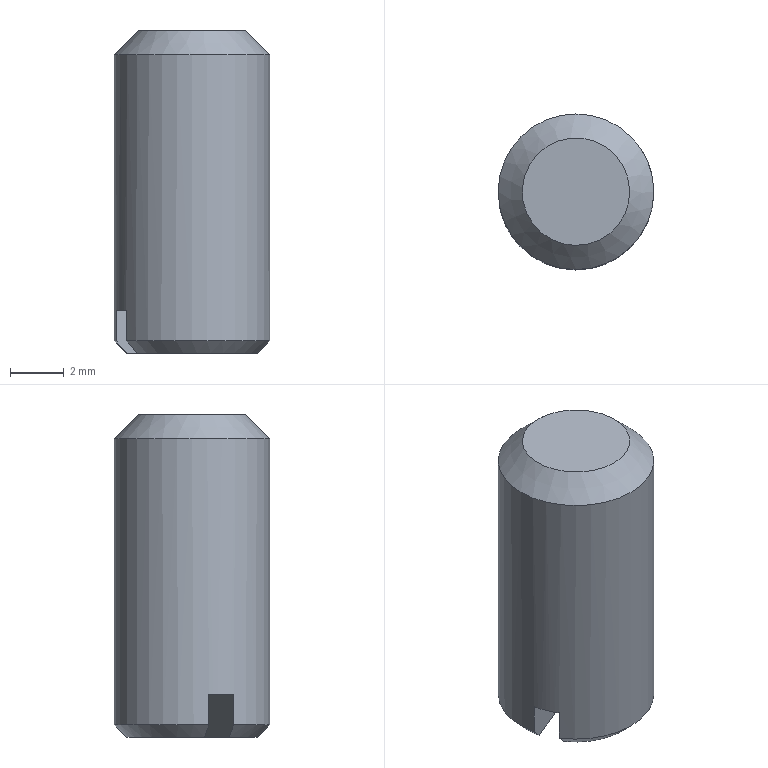Component | NX | GB73-85_M6X12 | 1 solid | 10 faces | box 5.8 x 5.8 x 12 mm | volume 299 mm3 | plane 6 | cone 3 | cylinder 1 | commonest cylinder face diameters 5.795 x1
STEP:
#1=CARTESIAN_POINT('',(0.,0.,0.));
#2=DIRECTION('',(0.,0.,1.));
#3=DIRECTION('',(1.,0.,0.));
#4=AXIS2_PLACEMENT_3D('',#1,#2,#3);
#5=CARTESIAN_POINT('',(-0.3824,57.675,-48.328));
#6=VERTEX_POINT('',#5);
#7=CARTESIAN_POINT('',(4.04,59.509,-48.328));
#8=VERTEX_POINT('',#7);
#9=CARTESIAN_POINT('',(-3.524,56.372,-48.328));
#10=DIRECTION('',(0.9237,0.383,0.));
#11=VECTOR('',#10,1.);
#12=LINE('',#9,#11);
#13=CARTESIAN_POINT('',(1.084,60.389,-48.328));
#14=DIRECTION('',(0.,0.,1.));
#15=DIRECTION('',(0.9237,0.383,0.));
#16=AXIS2_PLACEMENT_3D('',#13,#14,#15);
#17=PLANE('',#16);
#18=CARTESIAN_POINT('',(-5.795,-1.946));
#19=DIRECTION('',(1.,0.));
#20=VECTOR('',#19,1.);
#21=LINE('',#18,#20);
#22=(GEOMETRIC_REPRESENTATION_CONTEXT(2)PARAMETRIC_REPRESENTATION_CONTEXT()REPRESENTATION_CONTEXT('',''));
#23=DEFINITIONAL_REPRESENTATION('',(#21),#22);
#24=PCURVE('',#17,#23);
#25=CARTESIAN_POINT('',(-3.524,56.372,-48.328));
#26=DIRECTION('',(-0.383,0.9237,-0.));
#27=DIRECTION('',(0.,-0.,-1.));
#28=AXIS2_PLACEMENT_3D('',#25,#26,#27);
#29=PLANE('',#28);
#30=CARTESIAN_POINT('',(0.,0.));
#31=DIRECTION('',(0.,-1.));
#32=VECTOR('',#31,1.);
#33=LINE('',#30,#32);
#34=(GEOMETRIC_REPRESENTATION_CONTEXT(2)PARAMETRIC_REPRESENTATION_CONTEXT()REPRESENTATION_CONTEXT('',''));
#35=DEFINITIONAL_REPRESENTATION('',(#33),#34);
#36=PCURVE('',#29,#35);
#37=SURFACE_CURVE('',#12,(#24,#36),.PCURVE_S1.);
#38=EDGE_CURVE('',#6,#8,#37,.T.);
#39=ORIENTED_EDGE('',*,*,#38,.F.);
#40=CARTESIAN_POINT('',(2.02,58.13,-48.328));
#41=DIRECTION('',(0.,0.,-1.));
#42=DIRECTION('',(-0.9237,-0.383,0.));
#43=AXIS2_PLACEMENT_3D('',#40,#41,#42);
#44=CIRCLE('',#43,2.446);
#45=CARTESIAN_POINT('',(-2.446,-2.446));
#46=CARTESIAN_POINT('',(-2.446,1.79));
#47=CARTESIAN_POINT('',(1.223,-0.3276));
#48=CARTESIAN_POINT('',(4.891,-2.446));
#49=CARTESIAN_POINT('',(1.223,-4.563));
#50=CARTESIAN_POINT('',(-2.446,-6.681));
#51=CARTESIAN_POINT('',(-2.446,-2.446));
#52=(BOUNDED_CURVE()B_SPLINE_CURVE(2,(#45,#46,#47,#48,#49,#50,#51),.UNSPECIFIED.,.T.,.F.)B_SPLINE_CURVE_WITH_KNOTS((1,2,2,2,2,1),(-2.094,0.,2.094,4.189,6.283,8.378),.UNSPECIFIED.)CURVE()GEOMETRIC_REPRESENTATION_ITEM()RATIONAL_B_SPLINE_CURVE((1.,0.5,1.,0.5,1.,0.5,1.))REPRESENTATION_ITEM(''));
#53=(GEOMETRIC_REPRESENTATION_CONTEXT(2)PARAMETRIC_REPRESENTATION_CONTEXT()REPRESENTATION_CONTEXT('',''));
#54=DEFINITIONAL_REPRESENTATION('',(#52),#53);
#55=PCURVE('',#17,#54);
#56=CARTESIAN_POINT('',(2.02,58.13,-47.876));
#57=DIRECTION('',(0.,0.,1.));
#58=DIRECTION('',(0.9237,0.383,0.));
#59=AXIS2_PLACEMENT_3D('',#56,#57,#58);
#60=CONICAL_SURFACE('',#59,2.897,0.7854);
#61=CARTESIAN_POINT('',(3.142,-0.452));
#62=DIRECTION('',(-1.,0.));
#63=VECTOR('',#62,1.);
#64=LINE('',#61,#63);
#65=(GEOMETRIC_REPRESENTATION_CONTEXT(2)PARAMETRIC_REPRESENTATION_CONTEXT()REPRESENTATION_CONTEXT('',''));
#66=DEFINITIONAL_REPRESENTATION('',(#64),#65);
#67=PCURVE('',#60,#66);
#68=SURFACE_CURVE('',#44,(#55,#67),.PCURVE_S1.);
#69=EDGE_CURVE('',#6,#8,#68,.T.);
#70=ORIENTED_EDGE('',*,*,#69,.T.);
#71=EDGE_LOOP('',(#39,#70));
#72=FACE_BOUND('',#71,.T.);
#73=ADVANCED_FACE('',(#72),#17,.F.);
#74=CARTESIAN_POINT('',(-0.8075,57.499,-47.876));
#75=VERTEX_POINT('',#74);
#76=CARTESIAN_POINT('',(4.465,59.685,-47.876));
#77=VERTEX_POINT('',#76);
#78=CARTESIAN_POINT('',(2.02,58.13,-47.876));
#79=DIRECTION('',(0.,0.,-1.));
#80=DIRECTION('',(-0.9237,-0.383,0.));
#81=AXIS2_PLACEMENT_3D('',#78,#79,#80);
#82=CIRCLE('',#81,2.897);
#83=CARTESIAN_POINT('',(3.142,-0.));
#84=DIRECTION('',(-1.,0.));
#85=VECTOR('',#84,1.);
#86=LINE('',#83,#85);
#87=(GEOMETRIC_REPRESENTATION_CONTEXT(2)PARAMETRIC_REPRESENTATION_CONTEXT()REPRESENTATION_CONTEXT('',''));
#88=DEFINITIONAL_REPRESENTATION('',(#86),#87);
#89=PCURVE('',#60,#88);
#90=CARTESIAN_POINT('',(2.02,58.13,-48.328));
#91=DIRECTION('',(0.,0.,-1.));
#92=DIRECTION('',(-0.9237,-0.383,0.));
#93=AXIS2_PLACEMENT_3D('',#90,#91,#92);
#94=CYLINDRICAL_SURFACE('',#93,2.897);
#95=CARTESIAN_POINT('',(-0.,-0.452));
#96=DIRECTION('',(1.,0.));
#97=VECTOR('',#96,1.);
#98=LINE('',#95,#97);
#99=(GEOMETRIC_REPRESENTATION_CONTEXT(2)PARAMETRIC_REPRESENTATION_CONTEXT()REPRESENTATION_CONTEXT('',''));
#100=DEFINITIONAL_REPRESENTATION('',(#98),#99);
#101=PCURVE('',#94,#100);
#102=SURFACE_CURVE('',#82,(#89,#101),.PCURVE_S1.);
#103=EDGE_CURVE('',#75,#77,#102,.T.);
#104=ORIENTED_EDGE('',*,*,#103,.T.);
#105=CARTESIAN_POINT('',(4.465,59.685,-47.876));
#106=CARTESIAN_POINT('',(4.324,59.627,-48.027));
#107=CARTESIAN_POINT('',(4.182,59.568,-48.178));
#108=CARTESIAN_POINT('',(4.04,59.509,-48.328));
#109=B_SPLINE_CURVE_WITH_KNOTS('',3,(#105,#106,#107,#108),.UNSPECIFIED.,.F.,.F.,(4,4),(0.,1.),.PIECEWISE_BEZIER_KNOTS.);
#110=CARTESIAN_POINT('',(0.1734,-0.));
#111=CARTESIAN_POINT('',(0.2059,-0.452));
#112=B_SPLINE_CURVE_WITH_KNOTS('',1,(#110,#111),.UNSPECIFIED.,.F.,.F.,(2,2),(0.,1.),.PIECEWISE_BEZIER_KNOTS.);
#113=(GEOMETRIC_REPRESENTATION_CONTEXT(2)PARAMETRIC_REPRESENTATION_CONTEXT()REPRESENTATION_CONTEXT('',''));
#114=DEFINITIONAL_REPRESENTATION('',(#112),#113);
#115=PCURVE('',#60,#114);
#116=CARTESIAN_POINT('',(-0.452,-8.649));
#117=CARTESIAN_POINT('',(-0.3011,-8.496));
#118=CARTESIAN_POINT('',(-0.1504,-8.342));
#119=CARTESIAN_POINT('',(0.,-8.189));
#120=B_SPLINE_CURVE_WITH_KNOTS('',3,(#116,#117,#118,#119),.UNSPECIFIED.,.F.,.F.,(4,4),(0.,1.),.PIECEWISE_BEZIER_KNOTS.);
#121=(GEOMETRIC_REPRESENTATION_CONTEXT(2)PARAMETRIC_REPRESENTATION_CONTEXT()REPRESENTATION_CONTEXT('',''));
#122=DEFINITIONAL_REPRESENTATION('',(#120),#121);
#123=PCURVE('',#29,#122);
#124=SURFACE_CURVE('',#109,(#115,#123),.PCURVE_S1.);
#125=EDGE_CURVE('',#77,#8,#124,.T.);
#126=ORIENTED_EDGE('',*,*,#125,.T.);
#127=ORIENTED_EDGE('',*,*,#69,.F.);
#128=CARTESIAN_POINT('',(-0.3824,57.675,-48.328));
#129=CARTESIAN_POINT('',(-0.5243,57.616,-48.178));
#130=CARTESIAN_POINT('',(-0.666,57.558,-48.027));
#131=CARTESIAN_POINT('',(-0.8075,57.499,-47.876));
#132=B_SPLINE_CURVE_WITH_KNOTS('',3,(#128,#129,#130,#131),.UNSPECIFIED.,.F.,.F.,(4,4),(0.,1.),.PIECEWISE_BEZIER_KNOTS.);
#133=CARTESIAN_POINT('',(2.936,-0.452));
#134=CARTESIAN_POINT('',(2.968,0.));
#135=B_SPLINE_CURVE_WITH_KNOTS('',1,(#133,#134),.UNSPECIFIED.,.F.,.F.,(2,2),(0.,1.),.PIECEWISE_BEZIER_KNOTS.);
#136=(GEOMETRIC_REPRESENTATION_CONTEXT(2)PARAMETRIC_REPRESENTATION_CONTEXT()REPRESENTATION_CONTEXT('',''));
#137=DEFINITIONAL_REPRESENTATION('',(#135),#136);
#138=PCURVE('',#60,#137);
#139=CARTESIAN_POINT('',(0.,-3.401));
#140=CARTESIAN_POINT('',(-0.1504,-3.248));
#141=CARTESIAN_POINT('',(-0.3011,-3.094));
#142=CARTESIAN_POINT('',(-0.452,-2.941));
#143=B_SPLINE_CURVE_WITH_KNOTS('',3,(#139,#140,#141,#142),.UNSPECIFIED.,.F.,.F.,(4,4),(0.,1.),.PIECEWISE_BEZIER_KNOTS.);
#144=(GEOMETRIC_REPRESENTATION_CONTEXT(2)PARAMETRIC_REPRESENTATION_CONTEXT()REPRESENTATION_CONTEXT('',''));
#145=DEFINITIONAL_REPRESENTATION('',(#143),#144);
#146=PCURVE('',#29,#145);
#147=SURFACE_CURVE('',#132,(#138,#146),.PCURVE_S1.);
#148=EDGE_CURVE('',#6,#75,#147,.T.);
#149=ORIENTED_EDGE('',*,*,#148,.T.);
#150=EDGE_LOOP('',(#104,#126,#127,#149));
#151=FACE_BOUND('',#150,.T.);
#152=ADVANCED_FACE('',(#151),#60,.T.);
#153=CARTESIAN_POINT('',(4.423,58.585,-48.328));
#154=VERTEX_POINT('',#153);
#155=CARTESIAN_POINT('',(0.0006373,56.752,-48.328));
#156=VERTEX_POINT('',#155);
#157=CARTESIAN_POINT('',(2.02,58.13,-48.328));
#158=DIRECTION('',(0.,0.,-1.));
#159=DIRECTION('',(-0.9237,-0.383,0.));
#160=AXIS2_PLACEMENT_3D('',#157,#158,#159);
#161=CIRCLE('',#160,2.446);
#162=CARTESIAN_POINT('',(1.084,60.389,-48.328));
#163=DIRECTION('',(0.,0.,1.));
#164=DIRECTION('',(0.9237,0.383,0.));
#165=AXIS2_PLACEMENT_3D('',#162,#163,#164);
#166=PLANE('',#165);
#167=CARTESIAN_POINT('',(-2.446,-2.446));
#168=CARTESIAN_POINT('',(-2.446,1.79));
#169=CARTESIAN_POINT('',(1.223,-0.3276));
#170=CARTESIAN_POINT('',(4.891,-2.446));
#171=CARTESIAN_POINT('',(1.223,-4.563));
#172=CARTESIAN_POINT('',(-2.446,-6.681));
#173=CARTESIAN_POINT('',(-2.446,-2.446));
#174=(BOUNDED_CURVE()B_SPLINE_CURVE(2,(#167,#168,#169,#170,#171,#172,#173),.UNSPECIFIED.,.T.,.F.)B_SPLINE_CURVE_WITH_KNOTS((1,2,2,2,2,1),(-2.094,0.,2.094,4.189,6.283,8.378),.UNSPECIFIED.)CURVE()GEOMETRIC_REPRESENTATION_ITEM()RATIONAL_B_SPLINE_CURVE((1.,0.5,1.,0.5,1.,0.5,1.))REPRESENTATION_ITEM(''));
#175=(GEOMETRIC_REPRESENTATION_CONTEXT(2)PARAMETRIC_REPRESENTATION_CONTEXT()REPRESENTATION_CONTEXT('',''));
#176=DEFINITIONAL_REPRESENTATION('',(#174),#175);
#177=PCURVE('',#166,#176);
#178=CARTESIAN_POINT('',(2.02,58.13,-47.876));
#179=DIRECTION('',(0.,0.,1.));
#180=DIRECTION('',(0.9237,0.383,0.));
#181=AXIS2_PLACEMENT_3D('',#178,#179,#180);
#182=CONICAL_SURFACE('',#181,2.897,0.7854);
#183=CARTESIAN_POINT('',(9.425,-0.452));
#184=DIRECTION('',(-1.,0.));
#185=VECTOR('',#184,1.);
#186=LINE('',#183,#185);
#187=(GEOMETRIC_REPRESENTATION_CONTEXT(2)PARAMETRIC_REPRESENTATION_CONTEXT()REPRESENTATION_CONTEXT('',''));
#188=DEFINITIONAL_REPRESENTATION('',(#186),#187);
#189=PCURVE('',#182,#188);
#190=SURFACE_CURVE('',#161,(#177,#189),.PCURVE_S1.);
#191=EDGE_CURVE('',#154,#156,#190,.T.);
#192=ORIENTED_EDGE('',*,*,#191,.T.);
#193=CARTESIAN_POINT('',(-3.141,55.449,-48.328));
#194=DIRECTION('',(0.9237,0.383,0.));
#195=VECTOR('',#194,1.);
#196=LINE('',#193,#195);
#197=CARTESIAN_POINT('',(-5.795,-2.946));
#198=DIRECTION('',(1.,0.));
#199=VECTOR('',#198,1.);
#200=LINE('',#197,#199);
#201=(GEOMETRIC_REPRESENTATION_CONTEXT(2)PARAMETRIC_REPRESENTATION_CONTEXT()REPRESENTATION_CONTEXT('',''));
#202=DEFINITIONAL_REPRESENTATION('',(#200),#201);
#203=PCURVE('',#166,#202);
#204=CARTESIAN_POINT('',(-3.141,55.449,-46.728));
#205=DIRECTION('',(0.383,-0.9237,-0.));
#206=DIRECTION('',(0.,-0.,1.));
#207=AXIS2_PLACEMENT_3D('',#204,#205,#206);
#208=PLANE('',#207);
#209=CARTESIAN_POINT('',(-1.6,-0.));
#210=DIRECTION('',(0.,-1.));
#211=VECTOR('',#210,1.);
#212=LINE('',#209,#211);
#213=(GEOMETRIC_REPRESENTATION_CONTEXT(2)PARAMETRIC_REPRESENTATION_CONTEXT()REPRESENTATION_CONTEXT('',''));
#214=DEFINITIONAL_REPRESENTATION('',(#212),#213);
#215=PCURVE('',#208,#214);
#216=SURFACE_CURVE('',#196,(#203,#215),.PCURVE_S1.);
#217=EDGE_CURVE('',#156,#154,#216,.T.);
#218=ORIENTED_EDGE('',*,*,#217,.T.);
#219=EDGE_LOOP('',(#192,#218));
#220=FACE_BOUND('',#219,.T.);
#221=ADVANCED_FACE('',(#220),#166,.F.);
#222=CARTESIAN_POINT('',(4.848,58.762,-47.876));
#223=VERTEX_POINT('',#222);
#224=CARTESIAN_POINT('',(-0.4245,56.575,-47.876));
#225=VERTEX_POINT('',#224);
#226=CARTESIAN_POINT('',(2.02,58.13,-47.876));
#227=DIRECTION('',(0.,0.,-1.));
#228=DIRECTION('',(-0.9237,-0.383,0.));
#229=AXIS2_PLACEMENT_3D('',#226,#227,#228);
#230=CIRCLE('',#229,2.897);
#231=CARTESIAN_POINT('',(9.425,0.));
#232=DIRECTION('',(-1.,-0.));
#233=VECTOR('',#232,1.);
#234=LINE('',#231,#233);
#235=(GEOMETRIC_REPRESENTATION_CONTEXT(2)PARAMETRIC_REPRESENTATION_CONTEXT()REPRESENTATION_CONTEXT('',''));
#236=DEFINITIONAL_REPRESENTATION('',(#234),#235);
#237=PCURVE('',#182,#236);
#238=CARTESIAN_POINT('',(0.,-0.452));
#239=DIRECTION('',(1.,0.));
#240=VECTOR('',#239,1.);
#241=LINE('',#238,#240);
#242=(GEOMETRIC_REPRESENTATION_CONTEXT(2)PARAMETRIC_REPRESENTATION_CONTEXT()REPRESENTATION_CONTEXT('',''));
#243=DEFINITIONAL_REPRESENTATION('',(#241),#242);
#244=PCURVE('',#94,#243);
#245=SURFACE_CURVE('',#230,(#237,#244),.PCURVE_S1.);
#246=EDGE_CURVE('',#223,#225,#245,.T.);
#247=ORIENTED_EDGE('',*,*,#246,.T.);
#248=CARTESIAN_POINT('',(-0.4245,56.575,-47.876));
#249=CARTESIAN_POINT('',(-0.283,56.634,-48.027));
#250=CARTESIAN_POINT('',(-0.1413,56.693,-48.178));
#251=CARTESIAN_POINT('',(0.0006373,56.752,-48.328));
#252=B_SPLINE_CURVE_WITH_KNOTS('',3,(#248,#249,#250,#251),.UNSPECIFIED.,.F.,.F.,(4,4),(0.,1.),.PIECEWISE_BEZIER_KNOTS.);
#253=CARTESIAN_POINT('',(3.315,0.));
#254=CARTESIAN_POINT('',(3.348,-0.452));
#255=B_SPLINE_CURVE_WITH_KNOTS('',1,(#253,#254),.UNSPECIFIED.,.F.,.F.,(2,2),(0.,1.),.PIECEWISE_BEZIER_KNOTS.);
#256=(GEOMETRIC_REPRESENTATION_CONTEXT(2)PARAMETRIC_REPRESENTATION_CONTEXT()REPRESENTATION_CONTEXT('',''));
#257=DEFINITIONAL_REPRESENTATION('',(#255),#256);
#258=PCURVE('',#182,#257);
#259=CARTESIAN_POINT('',(-1.148,-2.941));
#260=CARTESIAN_POINT('',(-1.299,-3.094));
#261=CARTESIAN_POINT('',(-1.45,-3.248));
#262=CARTESIAN_POINT('',(-1.6,-3.401));
#263=B_SPLINE_CURVE_WITH_KNOTS('',3,(#259,#260,#261,#262),.UNSPECIFIED.,.F.,.F.,(4,4),(0.,1.),.PIECEWISE_BEZIER_KNOTS.);
#264=(GEOMETRIC_REPRESENTATION_CONTEXT(2)PARAMETRIC_REPRESENTATION_CONTEXT()REPRESENTATION_CONTEXT('',''));
#265=DEFINITIONAL_REPRESENTATION('',(#263),#264);
#266=PCURVE('',#208,#265);
#267=SURFACE_CURVE('',#252,(#258,#266),.PCURVE_S1.);
#268=EDGE_CURVE('',#225,#156,#267,.T.);
#269=ORIENTED_EDGE('',*,*,#268,.T.);
#270=ORIENTED_EDGE('',*,*,#191,.F.);
#271=CARTESIAN_POINT('',(4.423,58.585,-48.328));
#272=CARTESIAN_POINT('',(4.565,58.644,-48.178));
#273=CARTESIAN_POINT('',(4.707,58.703,-48.027));
#274=CARTESIAN_POINT('',(4.848,58.762,-47.876));
#275=B_SPLINE_CURVE_WITH_KNOTS('',3,(#271,#272,#273,#274),.UNSPECIFIED.,.F.,.F.,(4,4),(0.,1.),.PIECEWISE_BEZIER_KNOTS.);
#276=CARTESIAN_POINT('',(6.077,-0.452));
#277=CARTESIAN_POINT('',(6.11,-0.));
#278=B_SPLINE_CURVE_WITH_KNOTS('',1,(#276,#277),.UNSPECIFIED.,.F.,.F.,(2,2),(0.,1.),.PIECEWISE_BEZIER_KNOTS.);
#279=(GEOMETRIC_REPRESENTATION_CONTEXT(2)PARAMETRIC_REPRESENTATION_CONTEXT()REPRESENTATION_CONTEXT('',''));
#280=DEFINITIONAL_REPRESENTATION('',(#278),#279);
#281=PCURVE('',#182,#280);
#282=CARTESIAN_POINT('',(-1.6,-8.189));
#283=CARTESIAN_POINT('',(-1.45,-8.342));
#284=CARTESIAN_POINT('',(-1.299,-8.496));
#285=CARTESIAN_POINT('',(-1.148,-8.649));
#286=B_SPLINE_CURVE_WITH_KNOTS('',3,(#282,#283,#284,#285),.UNSPECIFIED.,.F.,.F.,(4,4),(0.,1.),.PIECEWISE_BEZIER_KNOTS.);
#287=(GEOMETRIC_REPRESENTATION_CONTEXT(2)PARAMETRIC_REPRESENTATION_CONTEXT()REPRESENTATION_CONTEXT('',''));
#288=DEFINITIONAL_REPRESENTATION('',(#286),#287);
#289=PCURVE('',#208,#288);
#290=SURFACE_CURVE('',#275,(#281,#289),.PCURVE_S1.);
#291=EDGE_CURVE('',#154,#223,#290,.T.);
#292=ORIENTED_EDGE('',*,*,#291,.T.);
#293=EDGE_LOOP('',(#247,#269,#270,#292));
#294=FACE_BOUND('',#293,.T.);
#295=ADVANCED_FACE('',(#294),#182,.T.);
#296=ORIENTED_EDGE('',*,*,#103,.F.);
#297=CARTESIAN_POINT('',(-0.8075,57.499,-46.728));
#298=VERTEX_POINT('',#297);
#299=CARTESIAN_POINT('',(-0.8075,57.499,-48.328));
#300=DIRECTION('',(0.,0.,1.));
#301=VECTOR('',#300,1.);
#302=LINE('',#299,#301);
#303=CARTESIAN_POINT('',(0.1734,0.));
#304=DIRECTION('',(0.,-1.));
#305=VECTOR('',#304,1.);
#306=LINE('',#303,#305);
#307=(GEOMETRIC_REPRESENTATION_CONTEXT(2)PARAMETRIC_REPRESENTATION_CONTEXT()REPRESENTATION_CONTEXT('',''));
#308=DEFINITIONAL_REPRESENTATION('',(#306),#307);
#309=PCURVE('',#94,#308);
#310=CARTESIAN_POINT('',(0.,-2.941));
#311=DIRECTION('',(-1.,-0.));
#312=VECTOR('',#311,1.);
#313=LINE('',#310,#312);
#314=(GEOMETRIC_REPRESENTATION_CONTEXT(2)PARAMETRIC_REPRESENTATION_CONTEXT()REPRESENTATION_CONTEXT('',''));
#315=DEFINITIONAL_REPRESENTATION('',(#313),#314);
#316=PCURVE('',#29,#315);
#317=SURFACE_CURVE('',#302,(#309,#316),.PCURVE_S1.);
#318=EDGE_CURVE('',#75,#298,#317,.T.);
#319=ORIENTED_EDGE('',*,*,#318,.T.);
#320=CARTESIAN_POINT('',(-0.6561,57.02,-46.728));
#321=VERTEX_POINT('',#320);
#322=CARTESIAN_POINT('',(2.02,58.13,-46.728));
#323=DIRECTION('',(0.,0.,1.));
#324=DIRECTION('',(0.9237,0.383,0.));
#325=AXIS2_PLACEMENT_3D('',#322,#323,#324);
#326=CIRCLE('',#325,2.897);
#327=CARTESIAN_POINT('',(3.142,-1.6));
#328=DIRECTION('',(-1.,0.));
#329=VECTOR('',#328,1.);
#330=LINE('',#327,#329);
#331=(GEOMETRIC_REPRESENTATION_CONTEXT(2)PARAMETRIC_REPRESENTATION_CONTEXT()REPRESENTATION_CONTEXT('',''));
#332=DEFINITIONAL_REPRESENTATION('',(#330),#331);
#333=PCURVE('',#94,#332);
#334=CARTESIAN_POINT('',(-3.333,55.911,-46.728));
#335=DIRECTION('',(0.,0.,1.));
#336=DIRECTION('',(0.9237,0.383,0.));
#337=AXIS2_PLACEMENT_3D('',#334,#335,#336);
#338=PLANE('',#337);
#339=CARTESIAN_POINT('',(5.795,0.));
#340=DIRECTION('',(1.,-0.));
#341=AXIS2_PLACEMENT_2D('',#339,#340);
#342=CIRCLE('',#341,2.897);
#343=(GEOMETRIC_REPRESENTATION_CONTEXT(2)PARAMETRIC_REPRESENTATION_CONTEXT()REPRESENTATION_CONTEXT('',''));
#344=DEFINITIONAL_REPRESENTATION('',(#342),#343);
#345=PCURVE('',#338,#344);
#346=SURFACE_CURVE('',#326,(#333,#345),.PCURVE_S1.);
#347=EDGE_CURVE('',#298,#321,#346,.T.);
#348=ORIENTED_EDGE('',*,*,#347,.T.);
#349=CARTESIAN_POINT('',(-0.6561,57.02,-37.225));
#350=VERTEX_POINT('',#349);
#351=CARTESIAN_POINT('',(-0.6561,57.02,-37.225));
#352=CARTESIAN_POINT('',(-0.6561,57.02,-46.728));
#353=B_SPLINE_CURVE_WITH_KNOTS('',1,(#351,#352),.UNSPECIFIED.,.F.,.F.,(2,2),(-11.102,-1.6),.PIECEWISE_BEZIER_KNOTS.);
#354=CARTESIAN_POINT('',(0.,0.));
#355=DIRECTION('',(0.,1.));
#356=VECTOR('',#355,1.);
#357=LINE('',#354,#356);
#358=(GEOMETRIC_REPRESENTATION_CONTEXT(2)PARAMETRIC_REPRESENTATION_CONTEXT()REPRESENTATION_CONTEXT('',''));
#359=DEFINITIONAL_REPRESENTATION('',(#357),#358);
#360=PCURVE('',#94,#359);
#361=CARTESIAN_POINT('',(6.283,0.));
#362=DIRECTION('',(0.,1.));
#363=VECTOR('',#362,1.);
#364=LINE('',#361,#363);
#365=(GEOMETRIC_REPRESENTATION_CONTEXT(2)PARAMETRIC_REPRESENTATION_CONTEXT()REPRESENTATION_CONTEXT('',''));
#366=DEFINITIONAL_REPRESENTATION('',(#364),#365);
#367=PCURVE('',#94,#366);
#368=SEAM_CURVE('',#353,(#360,#367),.PCURVE_S1.);
#369=EDGE_CURVE('',#350,#321,#368,.T.);
#370=ORIENTED_EDGE('',*,*,#369,.F.);
#371=CARTESIAN_POINT('',(2.02,58.13,-37.225));
#372=DIRECTION('',(0.,0.,-1.));
#373=DIRECTION('',(-0.9237,-0.383,0.));
#374=AXIS2_PLACEMENT_3D('',#371,#372,#373);
#375=CIRCLE('',#374,2.897);
#376=CARTESIAN_POINT('',(0.,-11.102));
#377=DIRECTION('',(1.,0.));
#378=VECTOR('',#377,1.);
#379=LINE('',#376,#378);
#380=(GEOMETRIC_REPRESENTATION_CONTEXT(2)PARAMETRIC_REPRESENTATION_CONTEXT()REPRESENTATION_CONTEXT('',''));
#381=DEFINITIONAL_REPRESENTATION('',(#379),#380);
#382=PCURVE('',#94,#381);
#383=CARTESIAN_POINT('',(2.02,58.13,-36.328));
#384=DIRECTION('',(0.,0.,-1.));
#385=DIRECTION('',(-0.9237,-0.383,0.));
#386=AXIS2_PLACEMENT_3D('',#383,#384,#385);
#387=CONICAL_SURFACE('',#386,2.,0.7854);
#388=CARTESIAN_POINT('',(0.,0.8975));
#389=DIRECTION('',(1.,0.));
#390=VECTOR('',#389,1.);
#391=LINE('',#388,#390);
#392=(GEOMETRIC_REPRESENTATION_CONTEXT(2)PARAMETRIC_REPRESENTATION_CONTEXT()REPRESENTATION_CONTEXT('',''));
#393=DEFINITIONAL_REPRESENTATION('',(#391),#392);
#394=PCURVE('',#387,#393);
#395=SURFACE_CURVE('',#375,(#382,#394),.PCURVE_S1.);
#396=EDGE_CURVE('',#350,#350,#395,.T.);
#397=ORIENTED_EDGE('',*,*,#396,.T.);
#398=ORIENTED_EDGE('',*,*,#369,.T.);
#399=CARTESIAN_POINT('',(-0.4245,56.575,-46.728));
#400=VERTEX_POINT('',#399);
#401=CARTESIAN_POINT('',(2.02,58.13,-46.728));
#402=DIRECTION('',(0.,0.,1.));
#403=DIRECTION('',(0.9237,0.383,0.));
#404=AXIS2_PLACEMENT_3D('',#401,#402,#403);
#405=CIRCLE('',#404,2.897);
#406=CARTESIAN_POINT('',(9.425,-1.6));
#407=DIRECTION('',(-1.,0.));
#408=VECTOR('',#407,1.);
#409=LINE('',#406,#408);
#410=(GEOMETRIC_REPRESENTATION_CONTEXT(2)PARAMETRIC_REPRESENTATION_CONTEXT()REPRESENTATION_CONTEXT('',''));
#411=DEFINITIONAL_REPRESENTATION('',(#409),#410);
#412=PCURVE('',#94,#411);
#413=CARTESIAN_POINT('',(5.795,0.));
#414=DIRECTION('',(1.,-0.));
#415=AXIS2_PLACEMENT_2D('',#413,#414);
#416=CIRCLE('',#415,2.897);
#417=(GEOMETRIC_REPRESENTATION_CONTEXT(2)PARAMETRIC_REPRESENTATION_CONTEXT()REPRESENTATION_CONTEXT('',''));
#418=DEFINITIONAL_REPRESENTATION('',(#416),#417);
#419=PCURVE('',#338,#418);
#420=SURFACE_CURVE('',#405,(#412,#419),.PCURVE_S1.);
#421=EDGE_CURVE('',#321,#400,#420,.T.);
#422=ORIENTED_EDGE('',*,*,#421,.T.);
#423=CARTESIAN_POINT('',(-0.4245,56.575,-48.328));
#424=DIRECTION('',(0.,0.,-1.));
#425=VECTOR('',#424,1.);
#426=LINE('',#423,#425);
#427=CARTESIAN_POINT('',(6.11,0.));
#428=DIRECTION('',(0.,1.));
#429=VECTOR('',#428,1.);
#430=LINE('',#427,#429);
#431=(GEOMETRIC_REPRESENTATION_CONTEXT(2)PARAMETRIC_REPRESENTATION_CONTEXT()REPRESENTATION_CONTEXT('',''));
#432=DEFINITIONAL_REPRESENTATION('',(#430),#431);
#433=PCURVE('',#94,#432);
#434=CARTESIAN_POINT('',(-1.6,-2.941));
#435=DIRECTION('',(-1.,-0.));
#436=VECTOR('',#435,1.);
#437=LINE('',#434,#436);
#438=(GEOMETRIC_REPRESENTATION_CONTEXT(2)PARAMETRIC_REPRESENTATION_CONTEXT()REPRESENTATION_CONTEXT('',''));
#439=DEFINITIONAL_REPRESENTATION('',(#437),#438);
#440=PCURVE('',#208,#439);
#441=SURFACE_CURVE('',#426,(#433,#440),.PCURVE_S1.);
#442=EDGE_CURVE('',#400,#225,#441,.T.);
#443=ORIENTED_EDGE('',*,*,#442,.T.);
#444=ORIENTED_EDGE('',*,*,#246,.F.);
#445=CARTESIAN_POINT('',(4.848,58.762,-46.728));
#446=VERTEX_POINT('',#445);
#447=CARTESIAN_POINT('',(4.848,58.762,-48.328));
#448=DIRECTION('',(0.,0.,1.));
#449=VECTOR('',#448,1.);
#450=LINE('',#447,#449);
#451=CARTESIAN_POINT('',(3.315,0.));
#452=DIRECTION('',(0.,-1.));
#453=VECTOR('',#452,1.);
#454=LINE('',#451,#453);
#455=(GEOMETRIC_REPRESENTATION_CONTEXT(2)PARAMETRIC_REPRESENTATION_CONTEXT()REPRESENTATION_CONTEXT('',''));
#456=DEFINITIONAL_REPRESENTATION('',(#454),#455);
#457=PCURVE('',#94,#456);
#458=CARTESIAN_POINT('',(-1.6,-8.649));
#459=DIRECTION('',(1.,0.));
#460=VECTOR('',#459,1.);
#461=LINE('',#458,#460);
#462=(GEOMETRIC_REPRESENTATION_CONTEXT(2)PARAMETRIC_REPRESENTATION_CONTEXT()REPRESENTATION_CONTEXT('',''));
#463=DEFINITIONAL_REPRESENTATION('',(#461),#462);
#464=PCURVE('',#208,#463);
#465=SURFACE_CURVE('',#450,(#457,#464),.PCURVE_S1.);
#466=EDGE_CURVE('',#223,#446,#465,.T.);
#467=ORIENTED_EDGE('',*,*,#466,.T.);
#468=CARTESIAN_POINT('',(4.465,59.685,-46.728));
#469=VERTEX_POINT('',#468);
#470=CARTESIAN_POINT('',(2.02,58.13,-46.728));
#471=DIRECTION('',(0.,0.,1.));
#472=DIRECTION('',(0.9237,0.383,0.));
#473=AXIS2_PLACEMENT_3D('',#470,#471,#472);
#474=CIRCLE('',#473,2.897);
#475=CARTESIAN_POINT('',(9.425,-1.6));
#476=DIRECTION('',(-1.,0.));
#477=VECTOR('',#476,1.);
#478=LINE('',#475,#477);
#479=(GEOMETRIC_REPRESENTATION_CONTEXT(2)PARAMETRIC_REPRESENTATION_CONTEXT()REPRESENTATION_CONTEXT('',''));
#480=DEFINITIONAL_REPRESENTATION('',(#478),#479);
#481=PCURVE('',#94,#480);
#482=CARTESIAN_POINT('',(5.795,0.));
#483=DIRECTION('',(1.,-0.));
#484=AXIS2_PLACEMENT_2D('',#482,#483);
#485=CIRCLE('',#484,2.897);
#486=(GEOMETRIC_REPRESENTATION_CONTEXT(2)PARAMETRIC_REPRESENTATION_CONTEXT()REPRESENTATION_CONTEXT('',''));
#487=DEFINITIONAL_REPRESENTATION('',(#485),#486);
#488=PCURVE('',#338,#487);
#489=SURFACE_CURVE('',#474,(#481,#488),.PCURVE_S1.);
#490=EDGE_CURVE('',#446,#469,#489,.T.);
#491=ORIENTED_EDGE('',*,*,#490,.T.);
#492=CARTESIAN_POINT('',(4.465,59.685,-48.328));
#493=DIRECTION('',(0.,0.,-1.));
#494=VECTOR('',#493,1.);
#495=LINE('',#492,#494);
#496=CARTESIAN_POINT('',(2.968,0.));
#497=DIRECTION('',(0.,1.));
#498=VECTOR('',#497,1.);
#499=LINE('',#496,#498);
#500=(GEOMETRIC_REPRESENTATION_CONTEXT(2)PARAMETRIC_REPRESENTATION_CONTEXT()REPRESENTATION_CONTEXT('',''));
#501=DEFINITIONAL_REPRESENTATION('',(#499),#500);
#502=PCURVE('',#94,#501);
#503=CARTESIAN_POINT('',(0.,-8.649));
#504=DIRECTION('',(1.,0.));
#505=VECTOR('',#504,1.);
#506=LINE('',#503,#505);
#507=(GEOMETRIC_REPRESENTATION_CONTEXT(2)PARAMETRIC_REPRESENTATION_CONTEXT()REPRESENTATION_CONTEXT('',''));
#508=DEFINITIONAL_REPRESENTATION('',(#506),#507);
#509=PCURVE('',#29,#508);
#510=SURFACE_CURVE('',#495,(#502,#509),.PCURVE_S1.);
#511=EDGE_CURVE('',#469,#77,#510,.T.);
#512=ORIENTED_EDGE('',*,*,#511,.T.);
#513=EDGE_LOOP('',(#296,#319,#348,#370,#397,#398,#422,#443,#444,#467,#491,#512));
#514=FACE_BOUND('',#513,.T.);
#515=ADVANCED_FACE('',(#514),#94,.T.);
#516=ORIENTED_EDGE('',*,*,#396,.F.);
#517=CARTESIAN_POINT('',(0.1729,57.364,-36.328));
#518=VERTEX_POINT('',#517);
#519=CARTESIAN_POINT('',(0.1729,57.364,-36.328));
#520=CARTESIAN_POINT('',(-0.6561,57.02,-37.225));
#521=B_SPLINE_CURVE_WITH_KNOTS('',1,(#519,#520),.UNSPECIFIED.,.F.,.F.,(2,2),(0.,1.269),.PIECEWISE_BEZIER_KNOTS.);
#522=CARTESIAN_POINT('',(0.,0.));
#523=DIRECTION('',(0.,1.));
#524=VECTOR('',#523,1.);
#525=LINE('',#522,#524);
#526=(GEOMETRIC_REPRESENTATION_CONTEXT(2)PARAMETRIC_REPRESENTATION_CONTEXT()REPRESENTATION_CONTEXT('',''));
#527=DEFINITIONAL_REPRESENTATION('',(#525),#526);
#528=PCURVE('',#387,#527);
#529=CARTESIAN_POINT('',(6.283,0.));
#530=DIRECTION('',(0.,1.));
#531=VECTOR('',#530,1.);
#532=LINE('',#529,#531);
#533=(GEOMETRIC_REPRESENTATION_CONTEXT(2)PARAMETRIC_REPRESENTATION_CONTEXT()REPRESENTATION_CONTEXT('',''));
#534=DEFINITIONAL_REPRESENTATION('',(#532),#533);
#535=PCURVE('',#387,#534);
#536=SEAM_CURVE('',#521,(#528,#535),.PCURVE_S1.);
#537=EDGE_CURVE('',#518,#350,#536,.T.);
#538=ORIENTED_EDGE('',*,*,#537,.F.);
#539=CARTESIAN_POINT('',(2.02,58.13,-36.328));
#540=DIRECTION('',(0.,0.,-1.));
#541=DIRECTION('',(-0.9237,-0.383,0.));
#542=AXIS2_PLACEMENT_3D('',#539,#540,#541);
#543=CIRCLE('',#542,2.);
#544=CARTESIAN_POINT('',(0.,0.));
#545=DIRECTION('',(1.,0.));
#546=VECTOR('',#545,1.);
#547=LINE('',#544,#546);
#548=(GEOMETRIC_REPRESENTATION_CONTEXT(2)PARAMETRIC_REPRESENTATION_CONTEXT()REPRESENTATION_CONTEXT('',''));
#549=DEFINITIONAL_REPRESENTATION('',(#547),#548);
#550=PCURVE('',#387,#549);
#551=CARTESIAN_POINT('',(2.02,58.13,-36.328));
#552=DIRECTION('',(0.,0.,-1.));
#553=DIRECTION('',(-0.9237,-0.383,0.));
#554=AXIS2_PLACEMENT_3D('',#551,#552,#553);
#555=PLANE('',#554);
#556=CARTESIAN_POINT('',(0.,0.));
#557=DIRECTION('',(1.,0.));
#558=AXIS2_PLACEMENT_2D('',#556,#557);
#559=CIRCLE('',#558,2.);
#560=(GEOMETRIC_REPRESENTATION_CONTEXT(2)PARAMETRIC_REPRESENTATION_CONTEXT()REPRESENTATION_CONTEXT('',''));
#561=DEFINITIONAL_REPRESENTATION('',(#559),#560);
#562=PCURVE('',#555,#561);
#563=SURFACE_CURVE('',#543,(#550,#562),.PCURVE_S1.);
#564=EDGE_CURVE('',#518,#518,#563,.T.);
#565=ORIENTED_EDGE('',*,*,#564,.T.);
#566=ORIENTED_EDGE('',*,*,#537,.T.);
#567=EDGE_LOOP('',(#516,#538,#565,#566));
#568=FACE_BOUND('',#567,.T.);
#569=ADVANCED_FACE('',(#568),#387,.T.);
#570=ORIENTED_EDGE('',*,*,#564,.F.);
#571=EDGE_LOOP('',(#570));
#572=FACE_BOUND('',#571,.T.);
#573=ADVANCED_FACE('',(#572),#555,.F.);
#574=ORIENTED_EDGE('',*,*,#511,.F.);
#575=CARTESIAN_POINT('',(-3.524,56.372,-46.728));
#576=DIRECTION('',(0.9237,0.383,0.));
#577=VECTOR('',#576,1.);
#578=LINE('',#575,#577);
#579=CARTESIAN_POINT('',(-1.6,-0.));
#580=DIRECTION('',(0.,-1.));
#581=VECTOR('',#580,1.);
#582=LINE('',#579,#581);
#583=(GEOMETRIC_REPRESENTATION_CONTEXT(2)PARAMETRIC_REPRESENTATION_CONTEXT()REPRESENTATION_CONTEXT('',''));
#584=DEFINITIONAL_REPRESENTATION('',(#582),#583);
#585=PCURVE('',#29,#584);
#586=CARTESIAN_POINT('',(-0.,0.5));
#587=DIRECTION('',(1.,0.));
#588=VECTOR('',#587,1.);
#589=LINE('',#586,#588);
#590=(GEOMETRIC_REPRESENTATION_CONTEXT(2)PARAMETRIC_REPRESENTATION_CONTEXT()REPRESENTATION_CONTEXT('',''));
#591=DEFINITIONAL_REPRESENTATION('',(#589),#590);
#592=PCURVE('',#338,#591);
#593=SURFACE_CURVE('',#578,(#585,#592),.PCURVE_S1.);
#594=EDGE_CURVE('',#298,#469,#593,.T.);
#595=ORIENTED_EDGE('',*,*,#594,.F.);
#596=ORIENTED_EDGE('',*,*,#318,.F.);
#597=ORIENTED_EDGE('',*,*,#148,.F.);
#598=ORIENTED_EDGE('',*,*,#38,.T.);
#599=ORIENTED_EDGE('',*,*,#125,.F.);
#600=EDGE_LOOP('',(#574,#595,#596,#597,#598,#599));
#601=FACE_BOUND('',#600,.T.);
#602=ADVANCED_FACE('',(#601),#29,.F.);
#603=ORIENTED_EDGE('',*,*,#421,.T.);
#604=CARTESIAN_POINT('',(-3.141,55.449,-46.728));
#605=DIRECTION('',(0.9237,0.383,0.));
#606=VECTOR('',#605,1.);
#607=LINE('',#604,#606);
#608=CARTESIAN_POINT('',(0.,-0.5));
#609=DIRECTION('',(1.,0.));
#610=VECTOR('',#609,1.);
#611=LINE('',#608,#610);
#612=(GEOMETRIC_REPRESENTATION_CONTEXT(2)PARAMETRIC_REPRESENTATION_CONTEXT()REPRESENTATION_CONTEXT('',''));
#613=DEFINITIONAL_REPRESENTATION('',(#611),#612);
#614=PCURVE('',#338,#613);
#615=CARTESIAN_POINT('',(0.,0.));
#616=DIRECTION('',(0.,-1.));
#617=VECTOR('',#616,1.);
#618=LINE('',#615,#617);
#619=(GEOMETRIC_REPRESENTATION_CONTEXT(2)PARAMETRIC_REPRESENTATION_CONTEXT()REPRESENTATION_CONTEXT('',''));
#620=DEFINITIONAL_REPRESENTATION('',(#618),#619);
#621=PCURVE('',#208,#620);
#622=SURFACE_CURVE('',#607,(#614,#621),.PCURVE_S1.);
#623=EDGE_CURVE('',#400,#446,#622,.T.);
#624=ORIENTED_EDGE('',*,*,#623,.T.);
#625=ORIENTED_EDGE('',*,*,#490,.T.);
#626=ORIENTED_EDGE('',*,*,#594,.F.);
#627=ORIENTED_EDGE('',*,*,#347,.T.);
#628=EDGE_LOOP('',(#603,#624,#625,#626,#627));
#629=FACE_BOUND('',#628,.F.);
#630=ADVANCED_FACE('',(#629),#338,.F.);
#631=ORIENTED_EDGE('',*,*,#442,.F.);
#632=ORIENTED_EDGE('',*,*,#623,.T.);
#633=ORIENTED_EDGE('',*,*,#466,.F.);
#634=ORIENTED_EDGE('',*,*,#291,.F.);
#635=ORIENTED_EDGE('',*,*,#217,.F.);
#636=ORIENTED_EDGE('',*,*,#268,.F.);
#637=EDGE_LOOP('',(#631,#632,#633,#634,#635,#636));
#638=FACE_BOUND('',#637,.T.);
#639=ADVANCED_FACE('',(#638),#208,.F.);
#640=CLOSED_SHELL('',(#73,#152,#221,#295,#515,#569,#573,#602,#630,#639));
#641=MANIFOLD_SOLID_BREP('',#640);
#642=(LENGTH_UNIT()NAMED_UNIT(*)SI_UNIT(.MILLI.,.METRE.));
#643=UNCERTAINTY_MEASURE_WITH_UNIT(LENGTH_MEASURE(0.002),#642,'','');
#644=(NAMED_UNIT(*)PLANE_ANGLE_UNIT()SI_UNIT($,.RADIAN.));
#645=(NAMED_UNIT(*)SI_UNIT($,.STERADIAN.)SOLID_ANGLE_UNIT());
#646=(GEOMETRIC_REPRESENTATION_CONTEXT(3)GLOBAL_UNCERTAINTY_ASSIGNED_CONTEXT((#643))GLOBAL_UNIT_ASSIGNED_CONTEXT((#642,#644,#645))REPRESENTATION_CONTEXT('',''));
#647=ADVANCED_BREP_SHAPE_REPRESENTATION('',(#4,#641),#646);